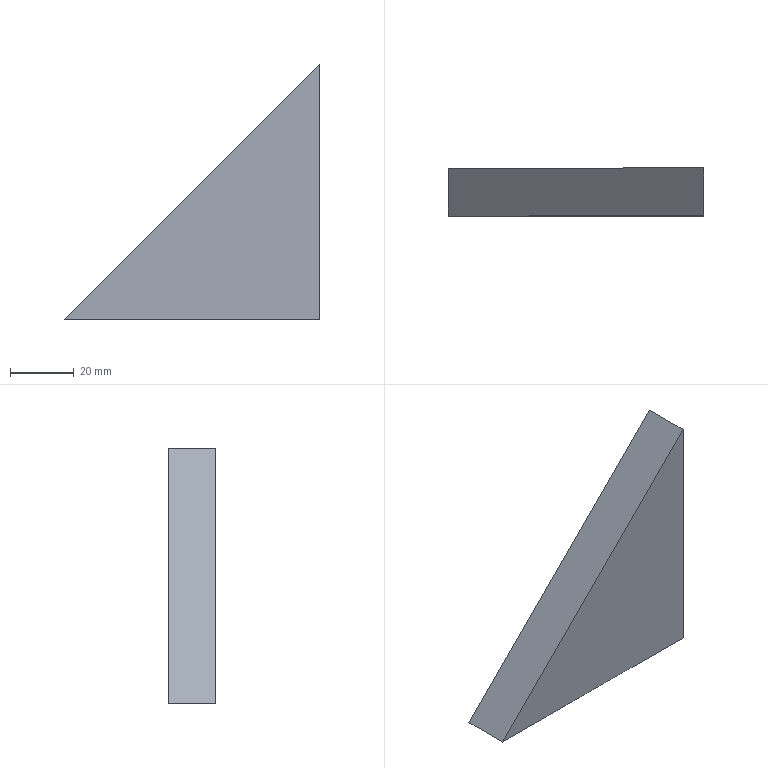Component | SolidWorks | STE21014.01-47-1 | 1 solid | 5 faces | box 80 x 15 x 80 mm | volume 48000 mm3 | plane 5 | material Q235
build123d program:
from build123d import *

# Parameters (mm, degrees)
BOSS_EXTRUDE1_DEPTH = 15


with BuildPart() as part:
    # Sketch1 → Boss-Extrude1 (new body)
    with BuildSketch(Plane(origin=(0, 0, 0), x_dir=(1, 0, 0), z_dir=(0, 1, 0))):
        Polygon((0, 0), (80, 0), (0, 80), align=None)
    extrude(amount=BOSS_EXTRUDE1_DEPTH)


solid = part.part

# Placed as in the assembly
solid = solid.moved(Location((265, 492.5, -550), (-180, 0, 180)))
STEP:
#1=COLOUR_RGB('',0.7922,0.8196,0.9333);
#2=FILL_AREA_STYLE_COLOUR('',#1);
#3=FILL_AREA_STYLE('',(#2));
#4=SURFACE_STYLE_FILL_AREA(#3);
#5=SURFACE_SIDE_STYLE('',(#4));
#6=SURFACE_STYLE_USAGE(.BOTH.,#5);
#7=PRESENTATION_STYLE_ASSIGNMENT((#6));
#8=CARTESIAN_POINT('',(7.283,19.98,-21.654));
#9=VERTEX_POINT('',#8);
#10=CARTESIAN_POINT('',(10.433,19.98,-21.654));
#11=VERTEX_POINT('',#10);
#12=CARTESIAN_POINT('',(10.433,19.98,-21.654));
#13=DIRECTION('',(1.,0.,0.));
#14=VECTOR('',#13,39.37);
#15=LINE('',#12,#14);
#16=EDGE_CURVE('',#9,#11,#15,.T.);
#17=ORIENTED_EDGE('',*,*,#16,.T.);
#18=CARTESIAN_POINT('',(10.433,19.39,-21.654));
#19=VERTEX_POINT('',#18);
#20=CARTESIAN_POINT('',(10.433,19.39,-21.654));
#21=DIRECTION('',(-0.,1.,-0.));
#22=VECTOR('',#21,39.37);
#23=LINE('',#20,#22);
#24=EDGE_CURVE('',#19,#11,#23,.T.);
#25=ORIENTED_EDGE('',*,*,#24,.F.);
#26=CARTESIAN_POINT('',(7.283,19.39,-21.654));
#27=VERTEX_POINT('',#26);
#28=CARTESIAN_POINT('',(10.433,19.39,-21.654));
#29=DIRECTION('',(1.,0.,0.));
#30=VECTOR('',#29,39.37);
#31=LINE('',#28,#30);
#32=EDGE_CURVE('',#27,#19,#31,.T.);
#33=ORIENTED_EDGE('',*,*,#32,.F.);
#34=CARTESIAN_POINT('',(7.283,19.39,-21.654));
#35=DIRECTION('',(-0.,1.,-0.));
#36=VECTOR('',#35,39.37);
#37=LINE('',#34,#36);
#38=EDGE_CURVE('',#27,#9,#37,.T.);
#39=ORIENTED_EDGE('',*,*,#38,.T.);
#40=EDGE_LOOP('',(#17,#25,#33,#39));
#41=FACE_OUTER_BOUND('',#40,.T.);
#42=CARTESIAN_POINT('',(10.433,19.39,-21.654));
#43=DIRECTION('',(-0.,0.,1.));
#44=DIRECTION('',(-1.,-0.,-0.));
#45=AXIS2_PLACEMENT_3D('',#42,#43,#44);
#46=PLANE('',#45);
#47=ADVANCED_FACE('',(#41),#46,.F.);
#48=CARTESIAN_POINT('',(10.433,19.98,-18.504));
#49=VERTEX_POINT('',#48);
#50=CARTESIAN_POINT('',(10.433,19.98,-21.654));
#51=DIRECTION('',(0.,0.,1.));
#52=VECTOR('',#51,39.37);
#53=LINE('',#50,#52);
#54=EDGE_CURVE('',#11,#49,#53,.T.);
#55=ORIENTED_EDGE('',*,*,#54,.T.);
#56=CARTESIAN_POINT('',(10.433,19.39,-18.504));
#57=VERTEX_POINT('',#56);
#58=CARTESIAN_POINT('',(10.433,19.39,-18.504));
#59=DIRECTION('',(-0.,1.,-0.));
#60=VECTOR('',#59,39.37);
#61=LINE('',#58,#60);
#62=EDGE_CURVE('',#57,#49,#61,.T.);
#63=ORIENTED_EDGE('',*,*,#62,.F.);
#64=CARTESIAN_POINT('',(10.433,19.39,-21.654));
#65=DIRECTION('',(0.,0.,1.));
#66=VECTOR('',#65,39.37);
#67=LINE('',#64,#66);
#68=EDGE_CURVE('',#19,#57,#67,.T.);
#69=ORIENTED_EDGE('',*,*,#68,.F.);
#70=ORIENTED_EDGE('',*,*,#24,.T.);
#71=EDGE_LOOP('',(#55,#63,#69,#70));
#72=FACE_OUTER_BOUND('',#71,.T.);
#73=CARTESIAN_POINT('',(10.433,19.39,-21.654));
#74=DIRECTION('',(-1.,-0.,0.));
#75=DIRECTION('',(-0.,-0.,-1.));
#76=AXIS2_PLACEMENT_3D('',#73,#74,#75);
#77=PLANE('',#76);
#78=ADVANCED_FACE('',(#72),#77,.F.);
#79=CARTESIAN_POINT('',(7.283,19.98,-21.654));
#80=DIRECTION('',(-0.7071,-0.,-0.7071));
#81=VECTOR('',#80,39.37);
#82=LINE('',#79,#81);
#83=EDGE_CURVE('',#49,#9,#82,.T.);
#84=ORIENTED_EDGE('',*,*,#83,.T.);
#85=ORIENTED_EDGE('',*,*,#38,.F.);
#86=CARTESIAN_POINT('',(7.283,19.39,-21.654));
#87=DIRECTION('',(-0.7071,-0.,-0.7071));
#88=VECTOR('',#87,39.37);
#89=LINE('',#86,#88);
#90=EDGE_CURVE('',#57,#27,#89,.T.);
#91=ORIENTED_EDGE('',*,*,#90,.F.);
#92=ORIENTED_EDGE('',*,*,#62,.T.);
#93=EDGE_LOOP('',(#84,#85,#91,#92));
#94=FACE_OUTER_BOUND('',#93,.T.);
#95=CARTESIAN_POINT('',(7.283,19.39,-21.654));
#96=DIRECTION('',(0.7071,0.,-0.7071));
#97=DIRECTION('',(0.7071,0.,0.7071));
#98=AXIS2_PLACEMENT_3D('',#95,#96,#97);
#99=PLANE('',#98);
#100=ADVANCED_FACE('',(#94),#99,.F.);
#101=ORIENTED_EDGE('',*,*,#32,.T.);
#102=ORIENTED_EDGE('',*,*,#68,.T.);
#103=ORIENTED_EDGE('',*,*,#90,.T.);
#104=EDGE_LOOP('',(#101,#102,#103));
#105=FACE_OUTER_BOUND('',#104,.T.);
#106=CARTESIAN_POINT('',(10.433,19.39,-21.654));
#107=DIRECTION('',(-0.,1.,-0.));
#108=DIRECTION('',(-1.,-0.,-0.));
#109=AXIS2_PLACEMENT_3D('',#106,#107,#108);
#110=PLANE('',#109);
#111=ADVANCED_FACE('',(#105),#110,.F.);
#112=ORIENTED_EDGE('',*,*,#16,.F.);
#113=ORIENTED_EDGE('',*,*,#83,.F.);
#114=ORIENTED_EDGE('',*,*,#54,.F.);
#115=EDGE_LOOP('',(#112,#113,#114));
#116=FACE_OUTER_BOUND('',#115,.T.);
#117=CARTESIAN_POINT('',(10.433,19.98,-21.654));
#118=DIRECTION('',(-0.,1.,-0.));
#119=DIRECTION('',(-1.,-0.,-0.));
#120=AXIS2_PLACEMENT_3D('',#117,#118,#119);
#121=PLANE('',#120);
#122=ADVANCED_FACE('',(#116),#121,.T.);
#123=CLOSED_SHELL('',(#47,#78,#100,#111,#122));
#124=MANIFOLD_SOLID_BREP('',#123);
#125=STYLED_ITEM('',(#7),#124);
#126=(LENGTH_UNIT()NAMED_UNIT(*)SI_UNIT($,.METRE.));
#127=LENGTH_MEASURE_WITH_UNIT(LENGTH_MEASURE(0.0254),#126);
#128=DIMENSIONAL_EXPONENTS(1.,0.,0.,0.,0.,0.,0.);
#129=(CONVERSION_BASED_UNIT('',#127)LENGTH_UNIT()NAMED_UNIT(#128));
#130=UNCERTAINTY_MEASURE_WITH_UNIT(LENGTH_MEASURE(0.00001),#129,'','');
#131=(NAMED_UNIT(*)PLANE_ANGLE_UNIT()SI_UNIT($,.RADIAN.));
#132=(NAMED_UNIT(*)SI_UNIT($,.STERADIAN.)SOLID_ANGLE_UNIT());
#133=(GEOMETRIC_REPRESENTATION_CONTEXT(3)GLOBAL_UNCERTAINTY_ASSIGNED_CONTEXT((#130))GLOBAL_UNIT_ASSIGNED_CONTEXT((#129,#131,#132))REPRESENTATION_CONTEXT('',''));
#134=MECHANICAL_DESIGN_GEOMETRIC_PRESENTATION_REPRESENTATION('',(#125),#133);
#135=CARTESIAN_POINT('',(0.,0.,0.));
#136=DIRECTION('',(0.,0.,1.));
#137=DIRECTION('',(1.,0.,0.));
#138=AXIS2_PLACEMENT_3D('',#135,#136,#137);
#139=(LENGTH_UNIT()NAMED_UNIT(*)SI_UNIT($,.METRE.));
#140=LENGTH_MEASURE_WITH_UNIT(LENGTH_MEASURE(0.0254),#139);
#141=DIMENSIONAL_EXPONENTS(1.,0.,0.,0.,0.,0.,0.);
#142=(CONVERSION_BASED_UNIT('',#140)LENGTH_UNIT()NAMED_UNIT(#141));
#143=UNCERTAINTY_MEASURE_WITH_UNIT(LENGTH_MEASURE(0.00001),#142,'','');
#144=(NAMED_UNIT(*)PLANE_ANGLE_UNIT()SI_UNIT($,.RADIAN.));
#145=(NAMED_UNIT(*)SI_UNIT($,.STERADIAN.)SOLID_ANGLE_UNIT());
#146=(GEOMETRIC_REPRESENTATION_CONTEXT(3)GLOBAL_UNCERTAINTY_ASSIGNED_CONTEXT((#143))GLOBAL_UNIT_ASSIGNED_CONTEXT((#142,#144,#145))REPRESENTATION_CONTEXT('',''));
#147=ADVANCED_BREP_SHAPE_REPRESENTATION('',(#124,#138),#146);
#148=PRESENTATION_LAYER_ASSIGNMENT('','',(#125));